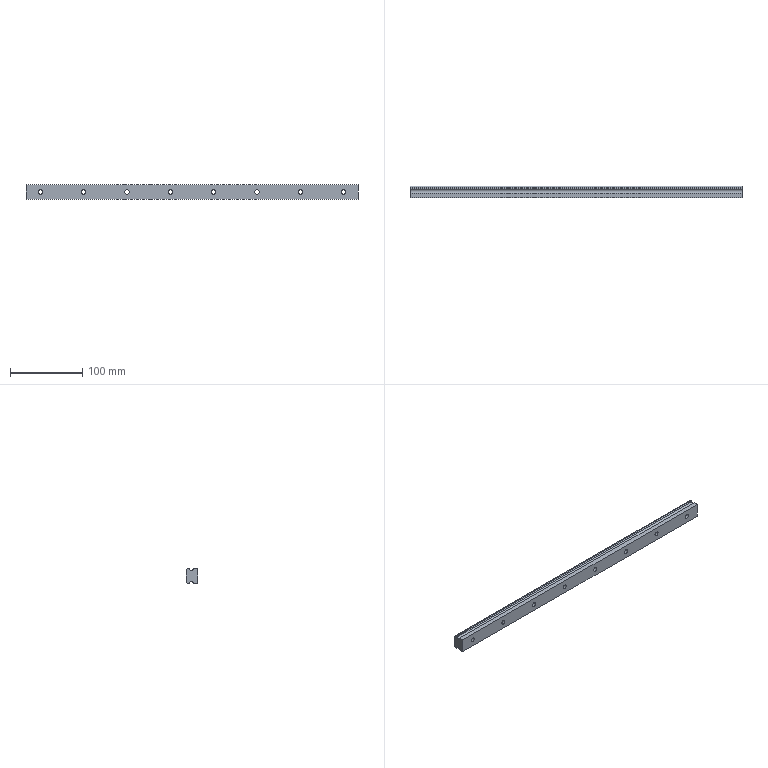Component | SolidWorks | SVR28-460-1_0MIM-SVR28-460-2-1 | 1 solid | 55 faces | box 460 x 15.5 x 20 mm | volume 125963 mm3 | cylinder 37 | plane 18 | commonest cylinder face diameters 6 x16 9.5 x16 5 x3 3 x2
build123d program:
from build123d import *

# Parameters (mm, degrees)
BOSS_EXTRUDE1_DEPTH      = 230
BOSS_EXTRUDE1_DEPTH_BACK = 230


with BuildPart() as part:
    # Sketch1 → Boss-Extrude1 (new, two sides: drawn at the far end of the back side and taken through both)
    with BuildSketch(Plane.XY.offset(-BOSS_EXTRUDE1_DEPTH_BACK)):
        with BuildLine():
            Line((-10, 0), (10, 0))
            Line((10, 0), (10, 6.18))
            ThreePointArc((10, 6.18), (7.546, 8.202), (9.062, 10.998))
            ThreePointArc((9.062, 10.998), (9.744, 11.55), (10, 12.388))
            Line((10, 12.388), (10, 14.043))
            Line((10, 14.043), (8.543, 15.5))
            Line((8.543, 15.5), (-8.543, 15.5))
            Line((-8.543, 15.5), (-10, 14.043))
            Line((-10, 14.043), (-10, 12.388))
            ThreePointArc((-10, 12.388), (-9.744, 11.55), (-9.062, 10.998))
            ThreePointArc((-9.062, 10.998), (-7.546, 8.202), (-10, 6.18))
            Line((-10, 6.18), (-10, 0))
        make_face()
    extrude(amount=BOSS_EXTRUDE1_DEPTH + BOSS_EXTRUDE1_DEPTH_BACK)

    # Sketch2 → Cut-Revolve1 (revolve, cut)
    with BuildSketch(Plane(origin=(0, 0, 0), x_dir=(0, 0, -1), z_dir=(1, 0, 0)), mode=Mode.PRIVATE) as cut_revolve1_sk:
        Polygon((210, 15.5), (214.75, 15.5), (214.75, 7), (213, 7), (213, 0), (210, 0), align=None)
    revolve(cut_revolve1_sk.sketch.rotate(Axis((0, 0, -210), (0, 1, 0)), 180), axis=Axis((0, 0, -210), (0, 1, 0)), mode=Mode.SUBTRACT)

    # Sketch3 → Cut-Revolve2 (revolve, cut)
    with BuildSketch(Plane(origin=(0, 0, 0), x_dir=(0, 0, -1), z_dir=(1, 0, 0)), mode=Mode.PRIVATE) as cut_revolve2_sk:
        Polygon((-210, 15.5), (-205.25, 15.5), (-205.25, 7), (-207, 7), (-207, 0), (-210, 0), align=None)
    revolve(cut_revolve2_sk.sketch.rotate(Axis((0, 0, 210), (0, 1, 0)), 180), axis=Axis((0, 0, 210), (0, 1, 0)), mode=Mode.SUBTRACT)

    # Sketch4 → Cut-Revolve3 (revolve, cut)
    with BuildSketch(Plane(origin=(0, 0, 0), x_dir=(0, 0, -1), z_dir=(1, 0, 0)), mode=Mode.PRIVATE) as cut_revolve3_sk:
        Polygon((-150, 15.5), (-145.25, 15.5), (-145.25, 7), (-147, 7), (-147, 0), (-150, 0), align=None)
    revolve(cut_revolve3_sk.sketch.rotate(Axis((0, 0, 150), (0, 1, 0)), 180), axis=Axis((0, 0, 150), (0, 1, 0)), mode=Mode.SUBTRACT)

    # Sketch5 → Cut-Revolve4 (revolve, cut)
    with BuildSketch(Plane(origin=(0, 0, 0), x_dir=(0, 0, -1), z_dir=(1, 0, 0)), mode=Mode.PRIVATE) as cut_revolve4_sk:
        Polygon((-90, 15.5), (-85.25, 15.5), (-85.25, 7), (-87, 7), (-87, 0), (-90, 0), align=None)
    revolve(cut_revolve4_sk.sketch.rotate(Axis((0, 0, 90), (0, 1, 0)), 180), axis=Axis((0, 0, 90), (0, 1, 0)), mode=Mode.SUBTRACT)

    # Sketch6 → Cut-Revolve5 (revolve, cut)
    with BuildSketch(Plane(origin=(0, 0, 0), x_dir=(0, 0, -1), z_dir=(1, 0, 0)), mode=Mode.PRIVATE) as cut_revolve5_sk:
        Polygon((-30, 15.5), (-25.25, 15.5), (-25.25, 7), (-27, 7), (-27, 0), (-30, 0), align=None)
    revolve(cut_revolve5_sk.sketch.rotate(Axis((0, 0, 30), (0, 1, 0)), 180), axis=Axis((0, 0, 30), (0, 1, 0)), mode=Mode.SUBTRACT)

    # Sketch7 → Cut-Revolve6 (revolve, cut)
    with BuildSketch(Plane(origin=(0, 0, 0), x_dir=(0, 0, -1), z_dir=(1, 0, 0)), mode=Mode.PRIVATE) as cut_revolve6_sk:
        Polygon((30, 15.5), (34.75, 15.5), (34.75, 7), (33, 7), (33, 0), (30, 0), align=None)
    revolve(cut_revolve6_sk.sketch.rotate(Axis((0, 0, -30), (0, 1, 0)), 180), axis=Axis((0, 0, -30), (0, 1, 0)), mode=Mode.SUBTRACT)

    # Sketch8 → Cut-Revolve7 (revolve, cut)
    with BuildSketch(Plane(origin=(0, 0, 0), x_dir=(0, 0, -1), z_dir=(1, 0, 0)), mode=Mode.PRIVATE) as cut_revolve7_sk:
        Polygon((90, 15.5), (94.75, 15.5), (94.75, 7), (93, 7), (93, 0), (90, 0), align=None)
    revolve(cut_revolve7_sk.sketch.rotate(Axis((0, 0, -90), (0, 1, 0)), 180), axis=Axis((0, 0, -90), (0, 1, 0)), mode=Mode.SUBTRACT)

    # Sketch9 → Cut-Revolve8 (revolve, cut)
    with BuildSketch(Plane(origin=(0, 0, 0), x_dir=(0, 0, -1), z_dir=(1, 0, 0)), mode=Mode.PRIVATE) as cut_revolve8_sk:
        Polygon((150, 15.5), (154.75, 15.5), (154.75, 7), (153, 7), (153, 0), (150, 0), align=None)
    revolve(cut_revolve8_sk.sketch.rotate(Axis((0, 0, -150), (0, 1, 0)), 180), axis=Axis((0, 0, -150), (0, 1, 0)), mode=Mode.SUBTRACT)


solid = part.part

# Placed as in the assembly
solid = solid.moved(Location((-97.009, 12.721, 94.589), (0, 90, 0)))